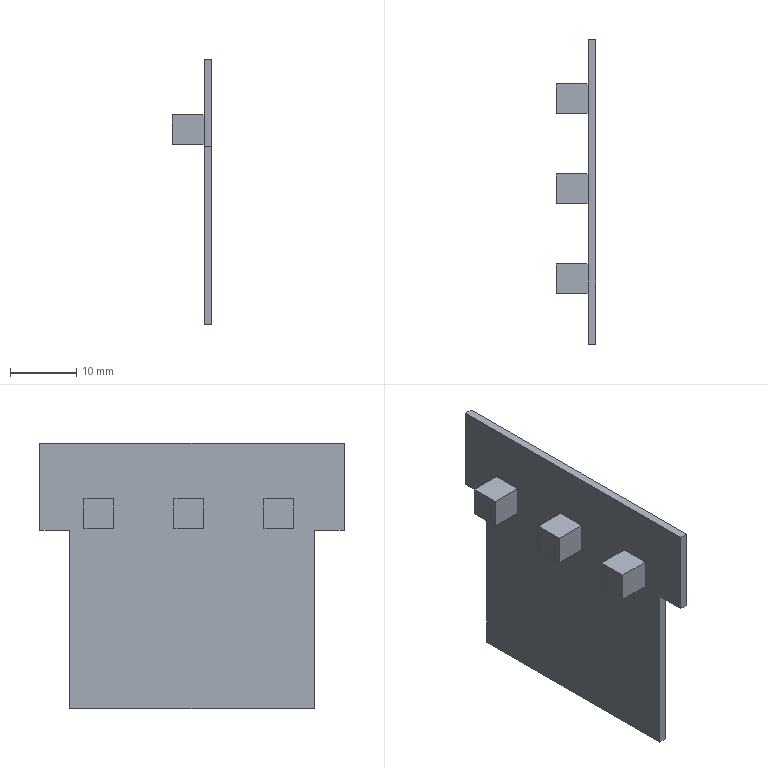Component | NX | PCB_SMALL | 1 solid | 25 faces | volume 2168 mm3 | plane 25